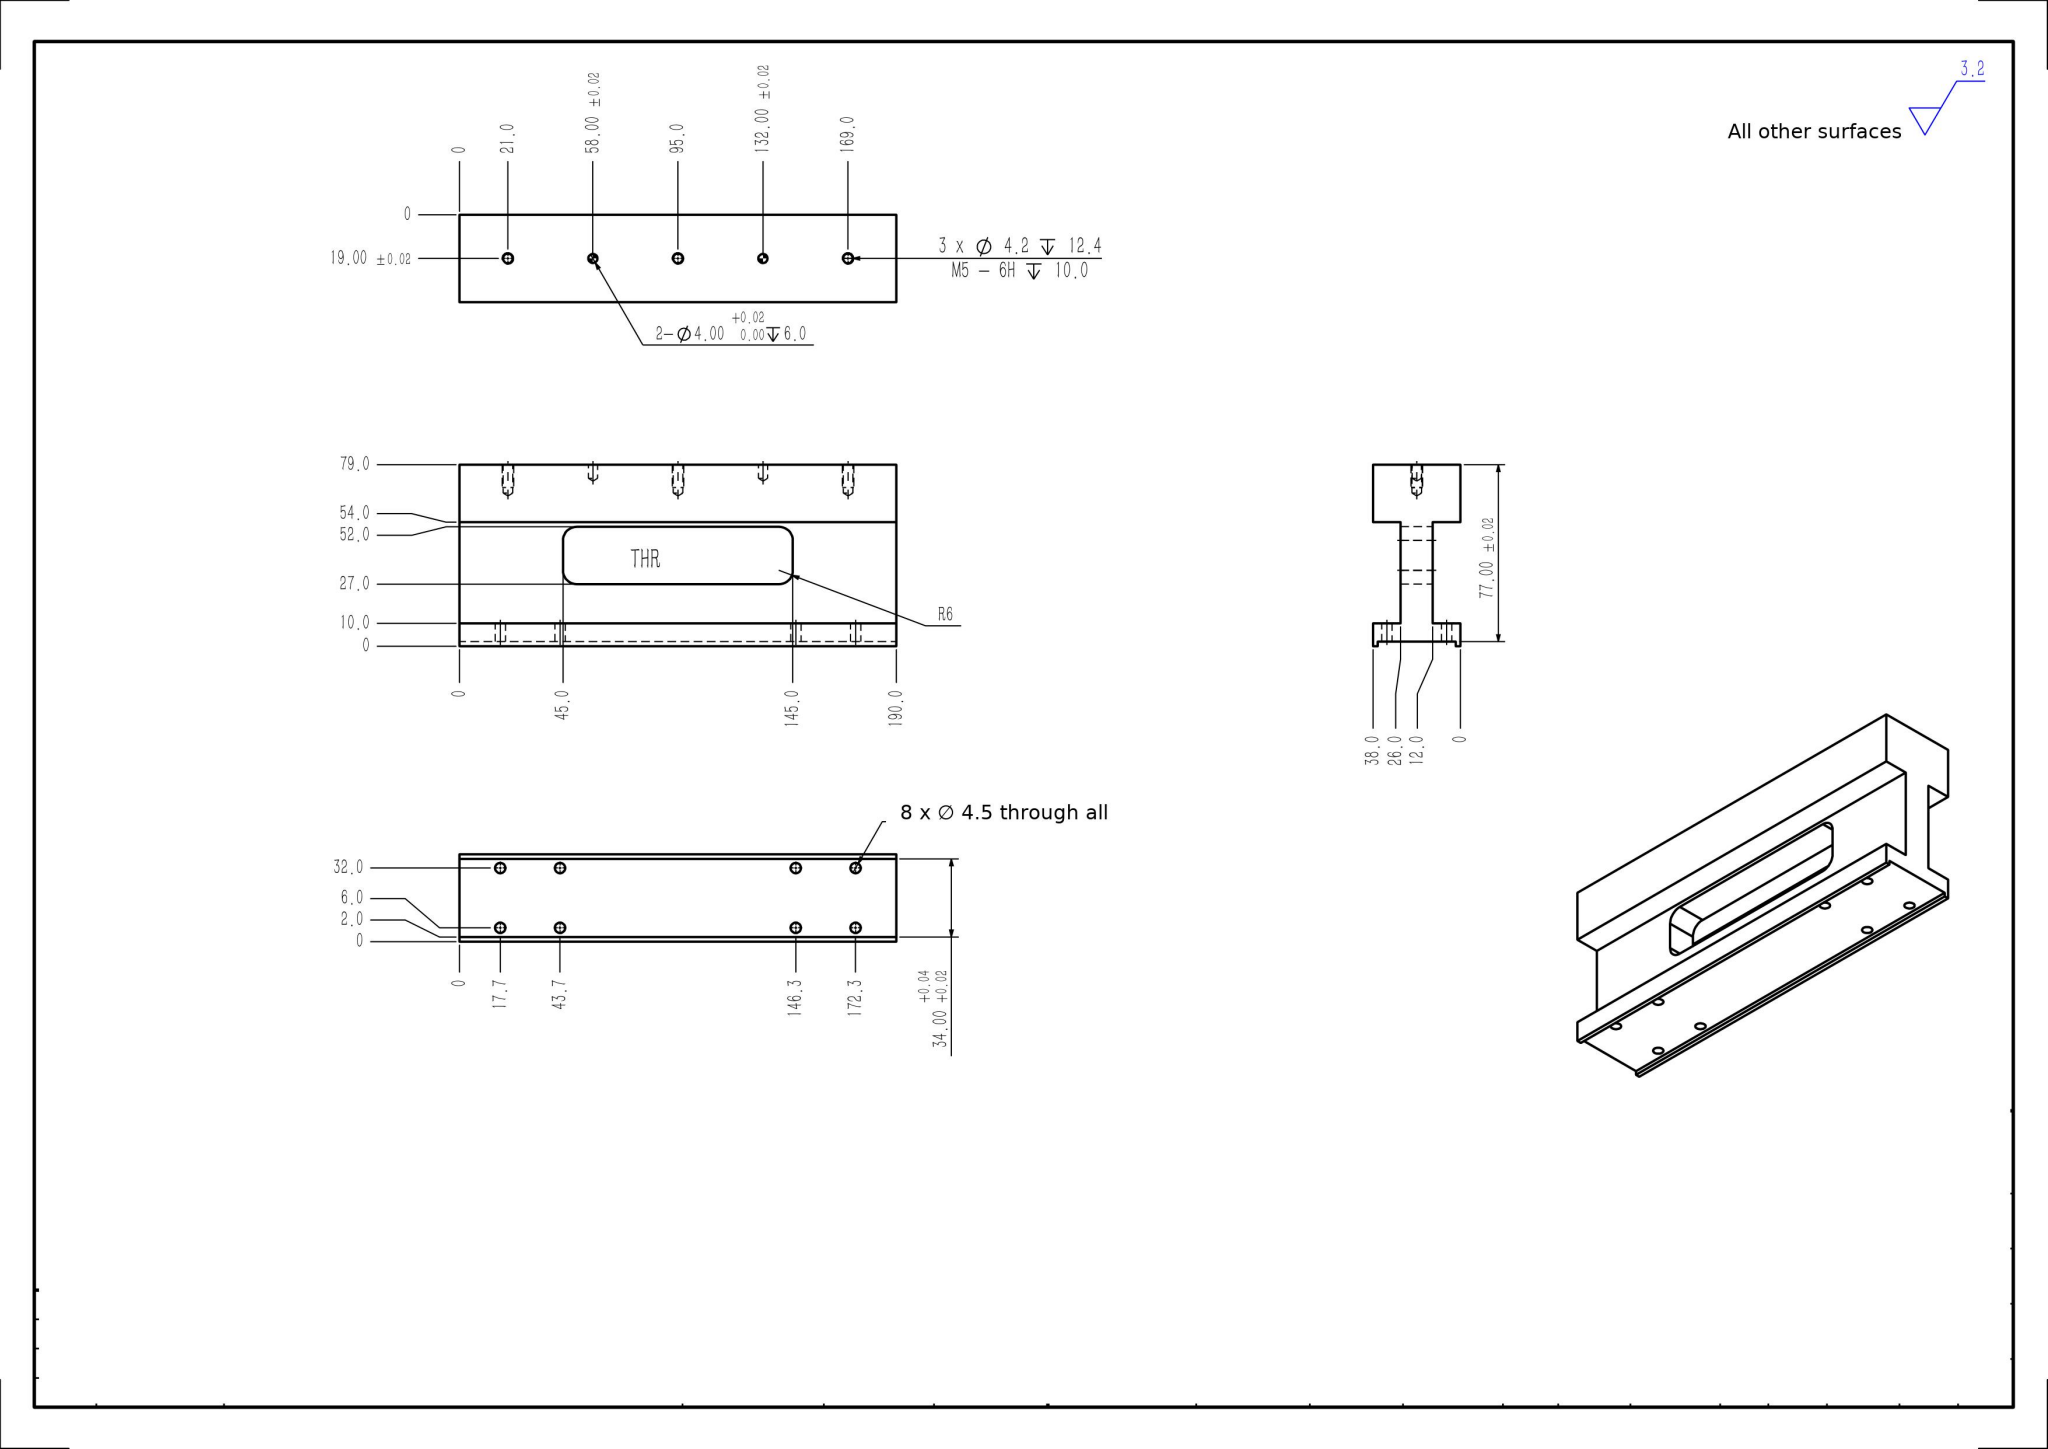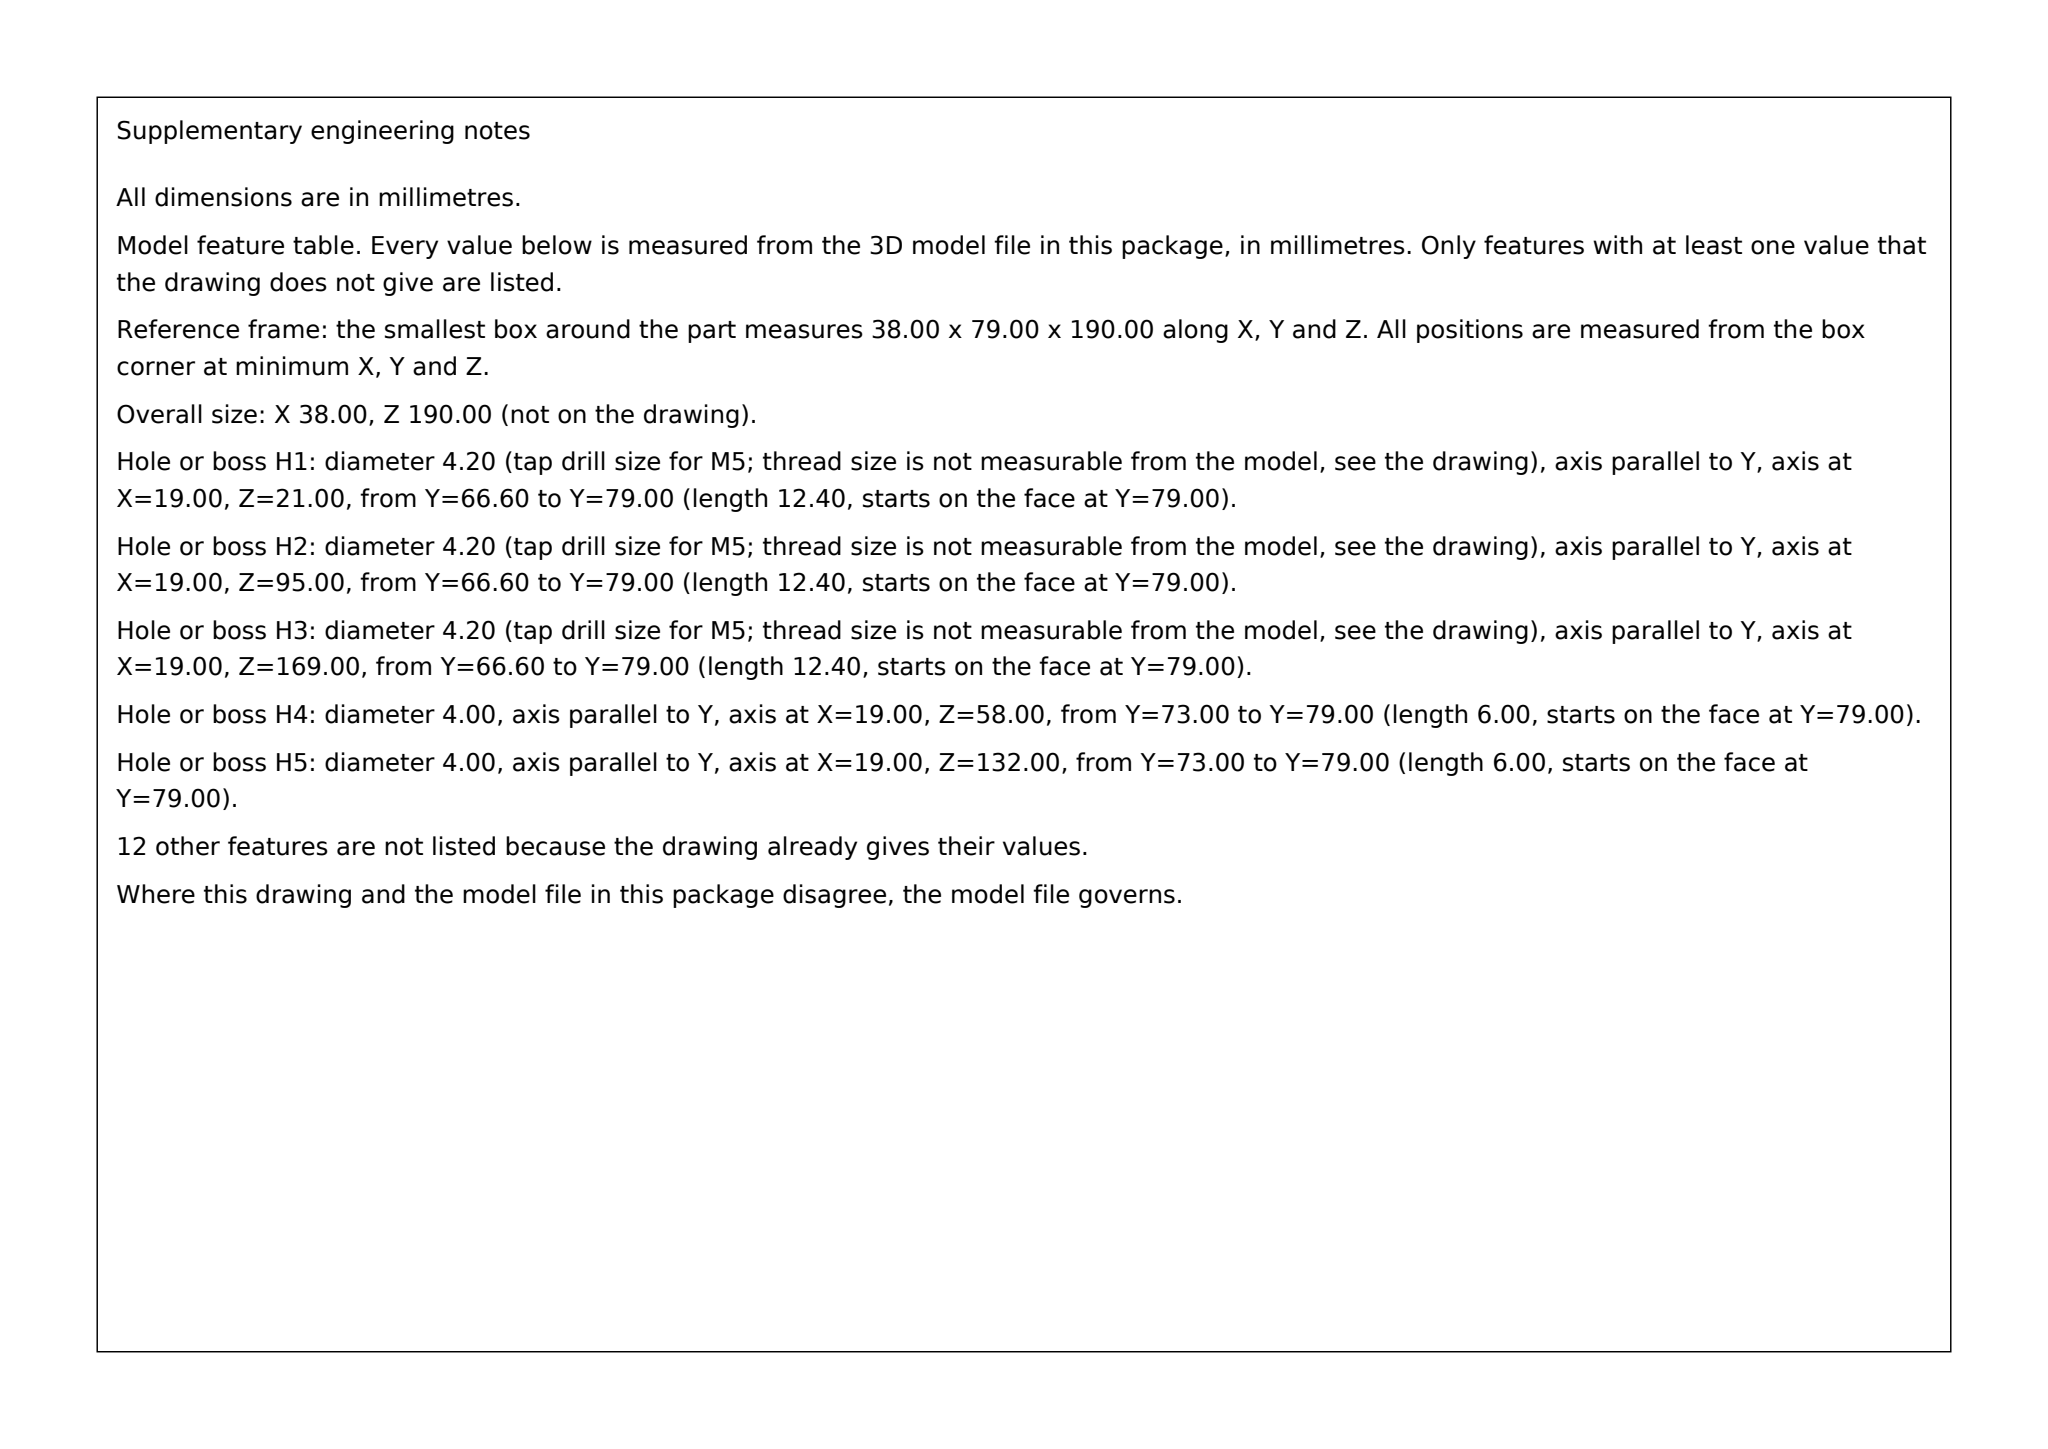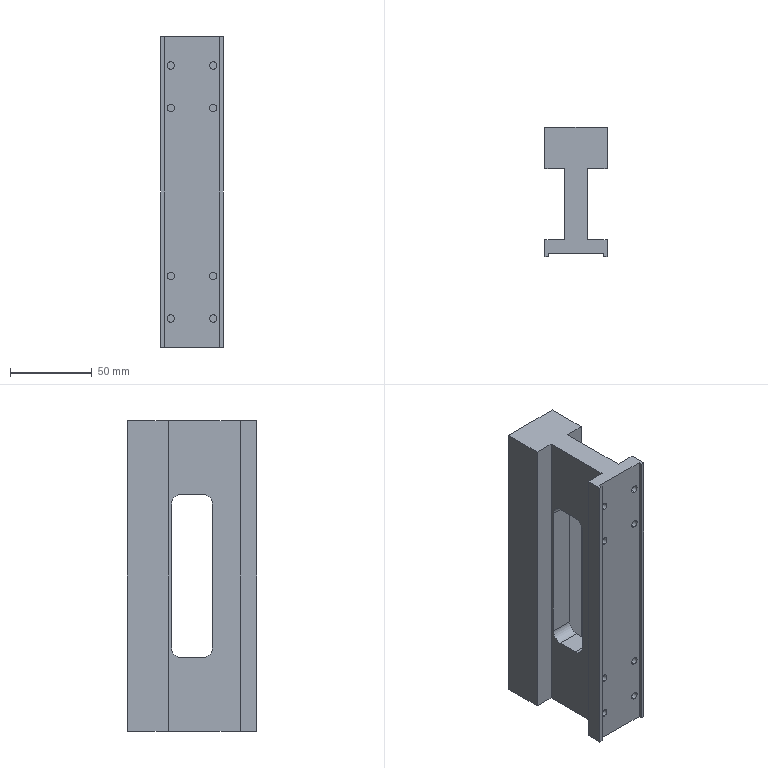Part | SolidWorks | mm | 1 solid | 62 faces | box 38 x 79 x 190 mm | volume 320541 mm3 | cylinder 30 | plane 22 | cone 10 | commonest cylinder face diameters 4.5 x16 4.2 x6 4 x4 12 x4
build123d program:
from build123d import *

# Parameters (mm, degrees)
BOSS_EXTRUDE1_DEPTH           = 95
SKETCH2_W                     = 12
SKETCH2_H                     = 44
CUT_EXTRUDE1_DEPTH            = 195.99
CUT_EXTRUDE2_DEPTH            = 107.119
M4_CLEARANCE_HOLE1_D          = 4.5
M4_CLEARANCE_HOLE1_DEPTH      = 10
M5_TAPPED_HOLE1_D             = 4.2
M5_TAPPED_HOLE1_DEPTH         = 12.4
M5_TAPPED_HOLE1_TIP           = 1.262
SIZE_MM_DOWEL_PIN_HOLE1_D     = 4
SIZE_MM_DOWEL_PIN_HOLE1_DEPTH = 6
SIZE_MM_DOWEL_PIN_HOLE1_TIP   = 1.202


with BuildPart() as part:
    # Sketch1 → Boss-Extrude1 (new, symmetric)
    with BuildSketch(Plane.XY):
        Polygon((-17, -39.5), (-17, -37.5), (17, -37.5), (17, -39.5), (19, -39.5), (19, 39.5), (-19, 39.5), (-19, -39.5), align=None)
    extrude(amount=BOSS_EXTRUDE1_DEPTH, both=True)

    # Sketch2 → Cut-Extrude1 (cut, through all)
    with BuildSketch(Plane.XY.offset(95)):
        with Locations((-13, -7.5)):
            Rectangle(SKETCH2_W, SKETCH2_H)
        with Locations((13, -7.5)):
            Rectangle(SKETCH2_W, SKETCH2_H)
    extrude(amount=-CUT_EXTRUDE1_DEPTH, mode=Mode.SUBTRACT)

    # Sketch3 → Cut-Extrude2 (cut, through all)
    with BuildSketch(Plane(origin=(7, 0, 0), x_dir=(0, 0, -1), z_dir=(1, 0, 0))):
        with BuildLine():
            Line((-44, -12.5), (44, -12.5))
            ThreePointArc((44, -12.5), (48.243, -10.743), (50, -6.5))
            Line((50, -6.5), (50, 6.5))
            ThreePointArc((50, 6.5), (48.243, 10.743), (44, 12.5))
            Line((44, 12.5), (-44, 12.5))
            ThreePointArc((-44, 12.5), (-48.243, 10.743), (-50, 6.5))
            Line((-50, 6.5), (-50, -6.5))
            ThreePointArc((-50, -6.5), (-48.243, -10.743), (-44, -12.5))
        make_face()
    extrude(amount=-CUT_EXTRUDE2_DEPTH, mode=Mode.SUBTRACT)

    # M4 Clearance Hole1
    with Locations(Plane(origin=(0, -29.5, 0), x_dir=(1, 0, 0), z_dir=(0, 1, 0))):
        with Locations((13, -77.3), (13, -51.3), (-13, -77.3), (-13, -51.3), (13, 51.3), (13, 77.3), (-13, 51.3), (-13, 77.3)):
            Hole(M4_CLEARANCE_HOLE1_D / 2, depth=M4_CLEARANCE_HOLE1_DEPTH)

    # M5 Tapped Hole1
    with Locations(Plane(origin=(0, 39.5, 0), x_dir=(1, 0, 0), z_dir=(0, 1, 0))):
        with Locations((0, 0), (0, 74), (0, -74)):
            Hole(M5_TAPPED_HOLE1_D / 2, depth=M5_TAPPED_HOLE1_DEPTH)
            with Locations((0, 0, -(M5_TAPPED_HOLE1_DEPTH + M5_TAPPED_HOLE1_TIP / 2))):  # 118° drill point
                Cone(0, M5_TAPPED_HOLE1_D / 2, M5_TAPPED_HOLE1_TIP, mode=Mode.SUBTRACT)

    # Size mm Dowel Pin Hole1
    with Locations(Plane(origin=(0, 39.5, 0), x_dir=(1, 0, 0), z_dir=(0, 1, 0))):
        with Locations((0, 37), (0, -37)):
            Hole(SIZE_MM_DOWEL_PIN_HOLE1_D / 2, depth=SIZE_MM_DOWEL_PIN_HOLE1_DEPTH)
            with Locations((0, 0, -(SIZE_MM_DOWEL_PIN_HOLE1_DEPTH + SIZE_MM_DOWEL_PIN_HOLE1_TIP / 2))):  # 118° drill point
                Cone(0, SIZE_MM_DOWEL_PIN_HOLE1_D / 2, SIZE_MM_DOWEL_PIN_HOLE1_TIP, mode=Mode.SUBTRACT)


solid = part.part